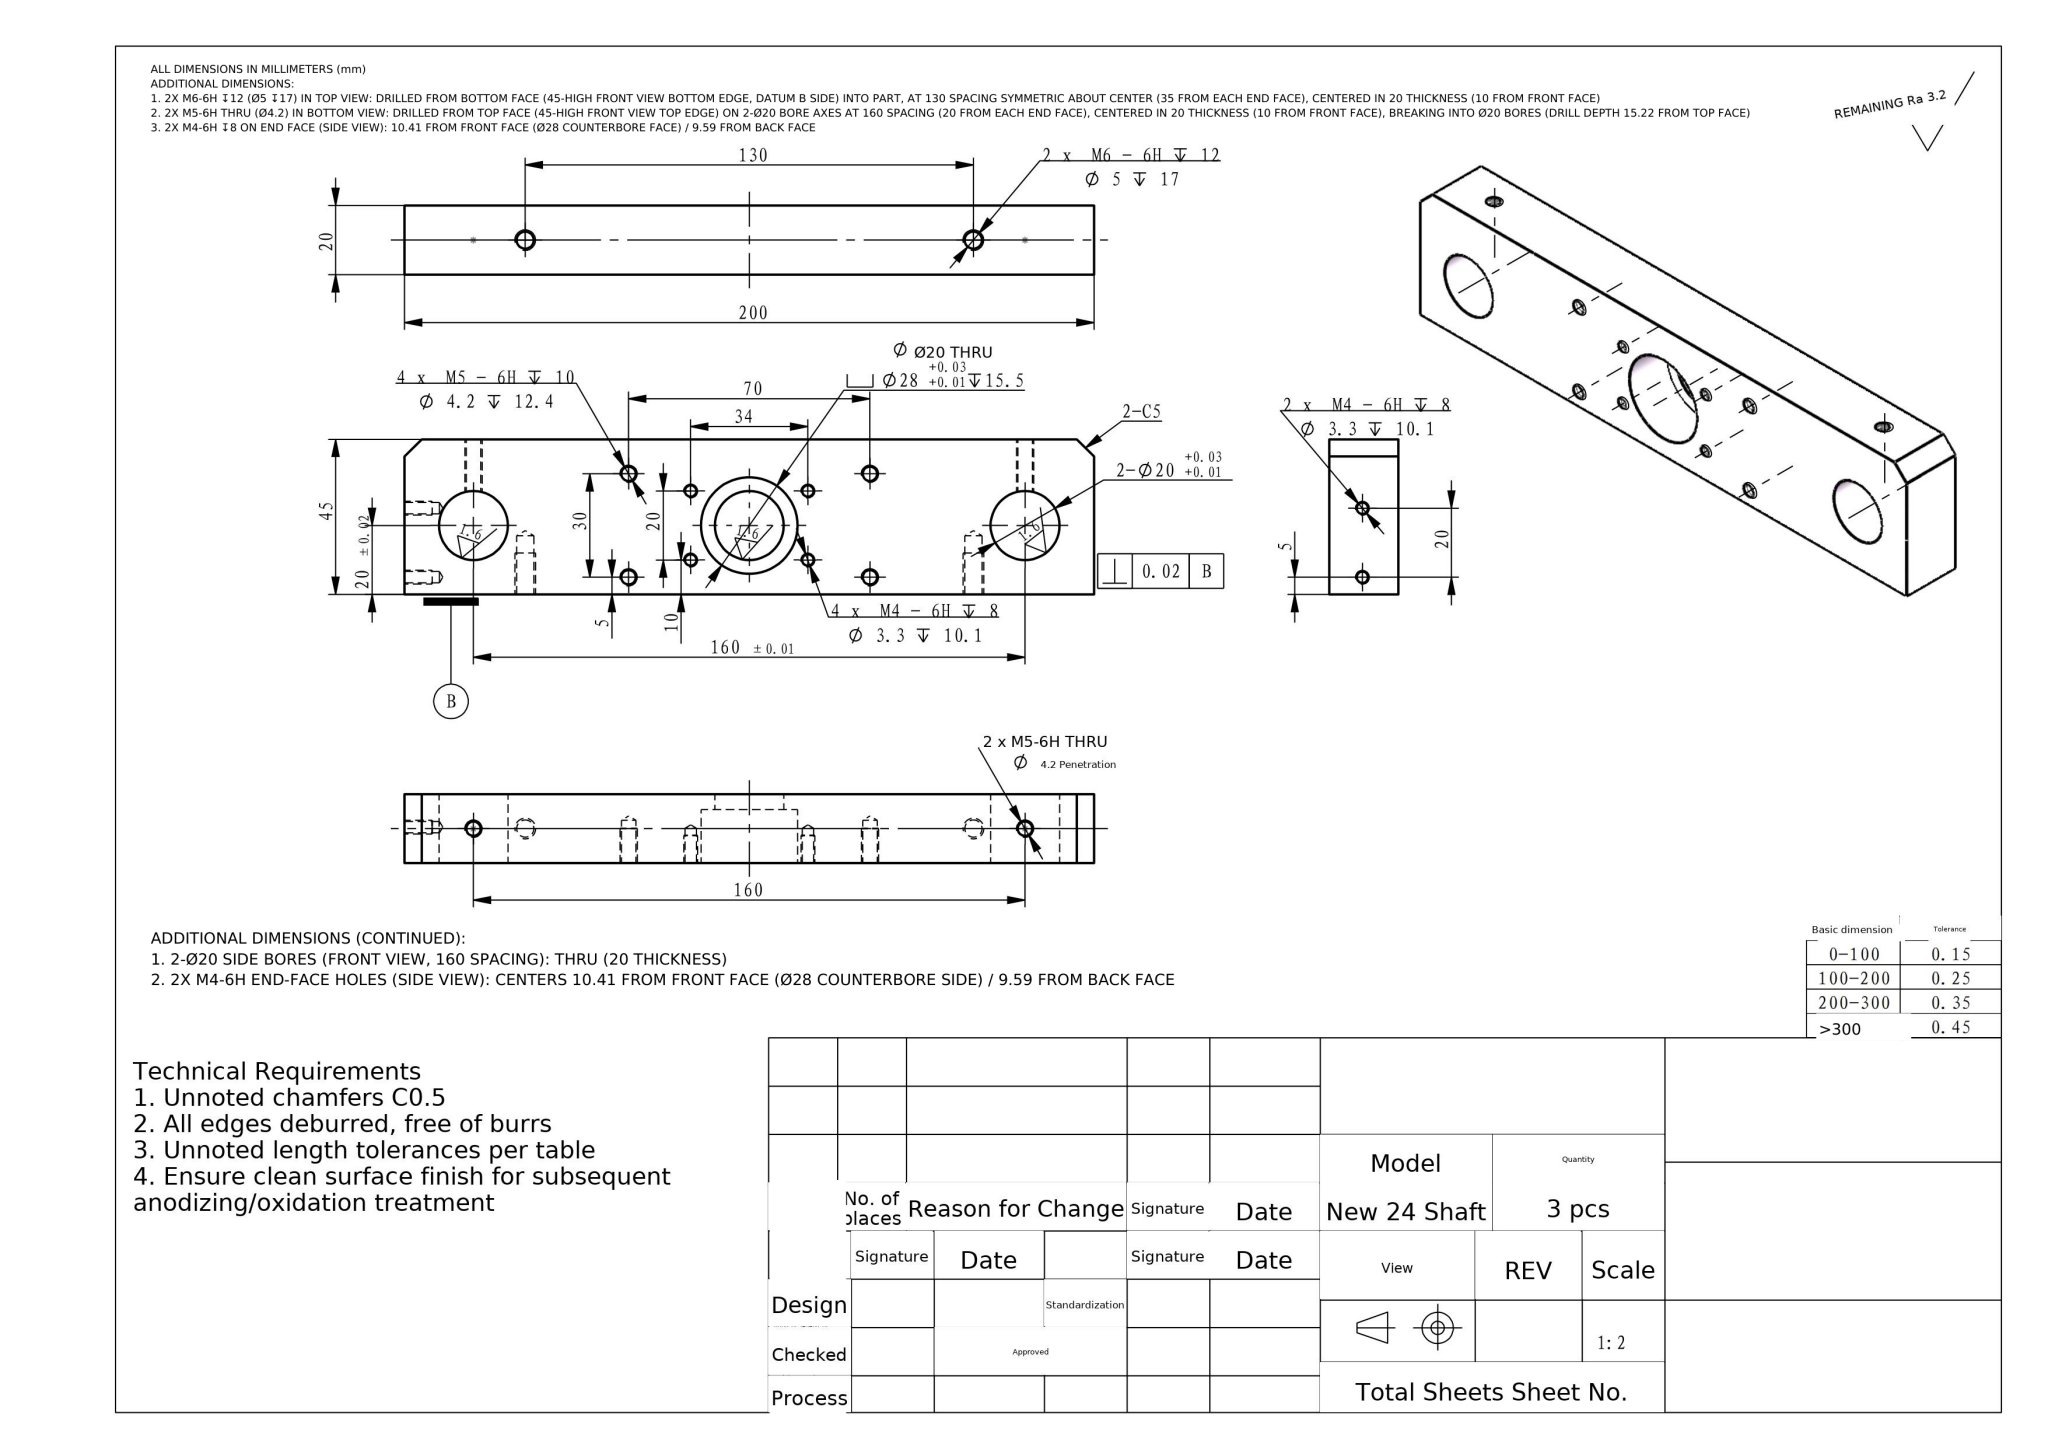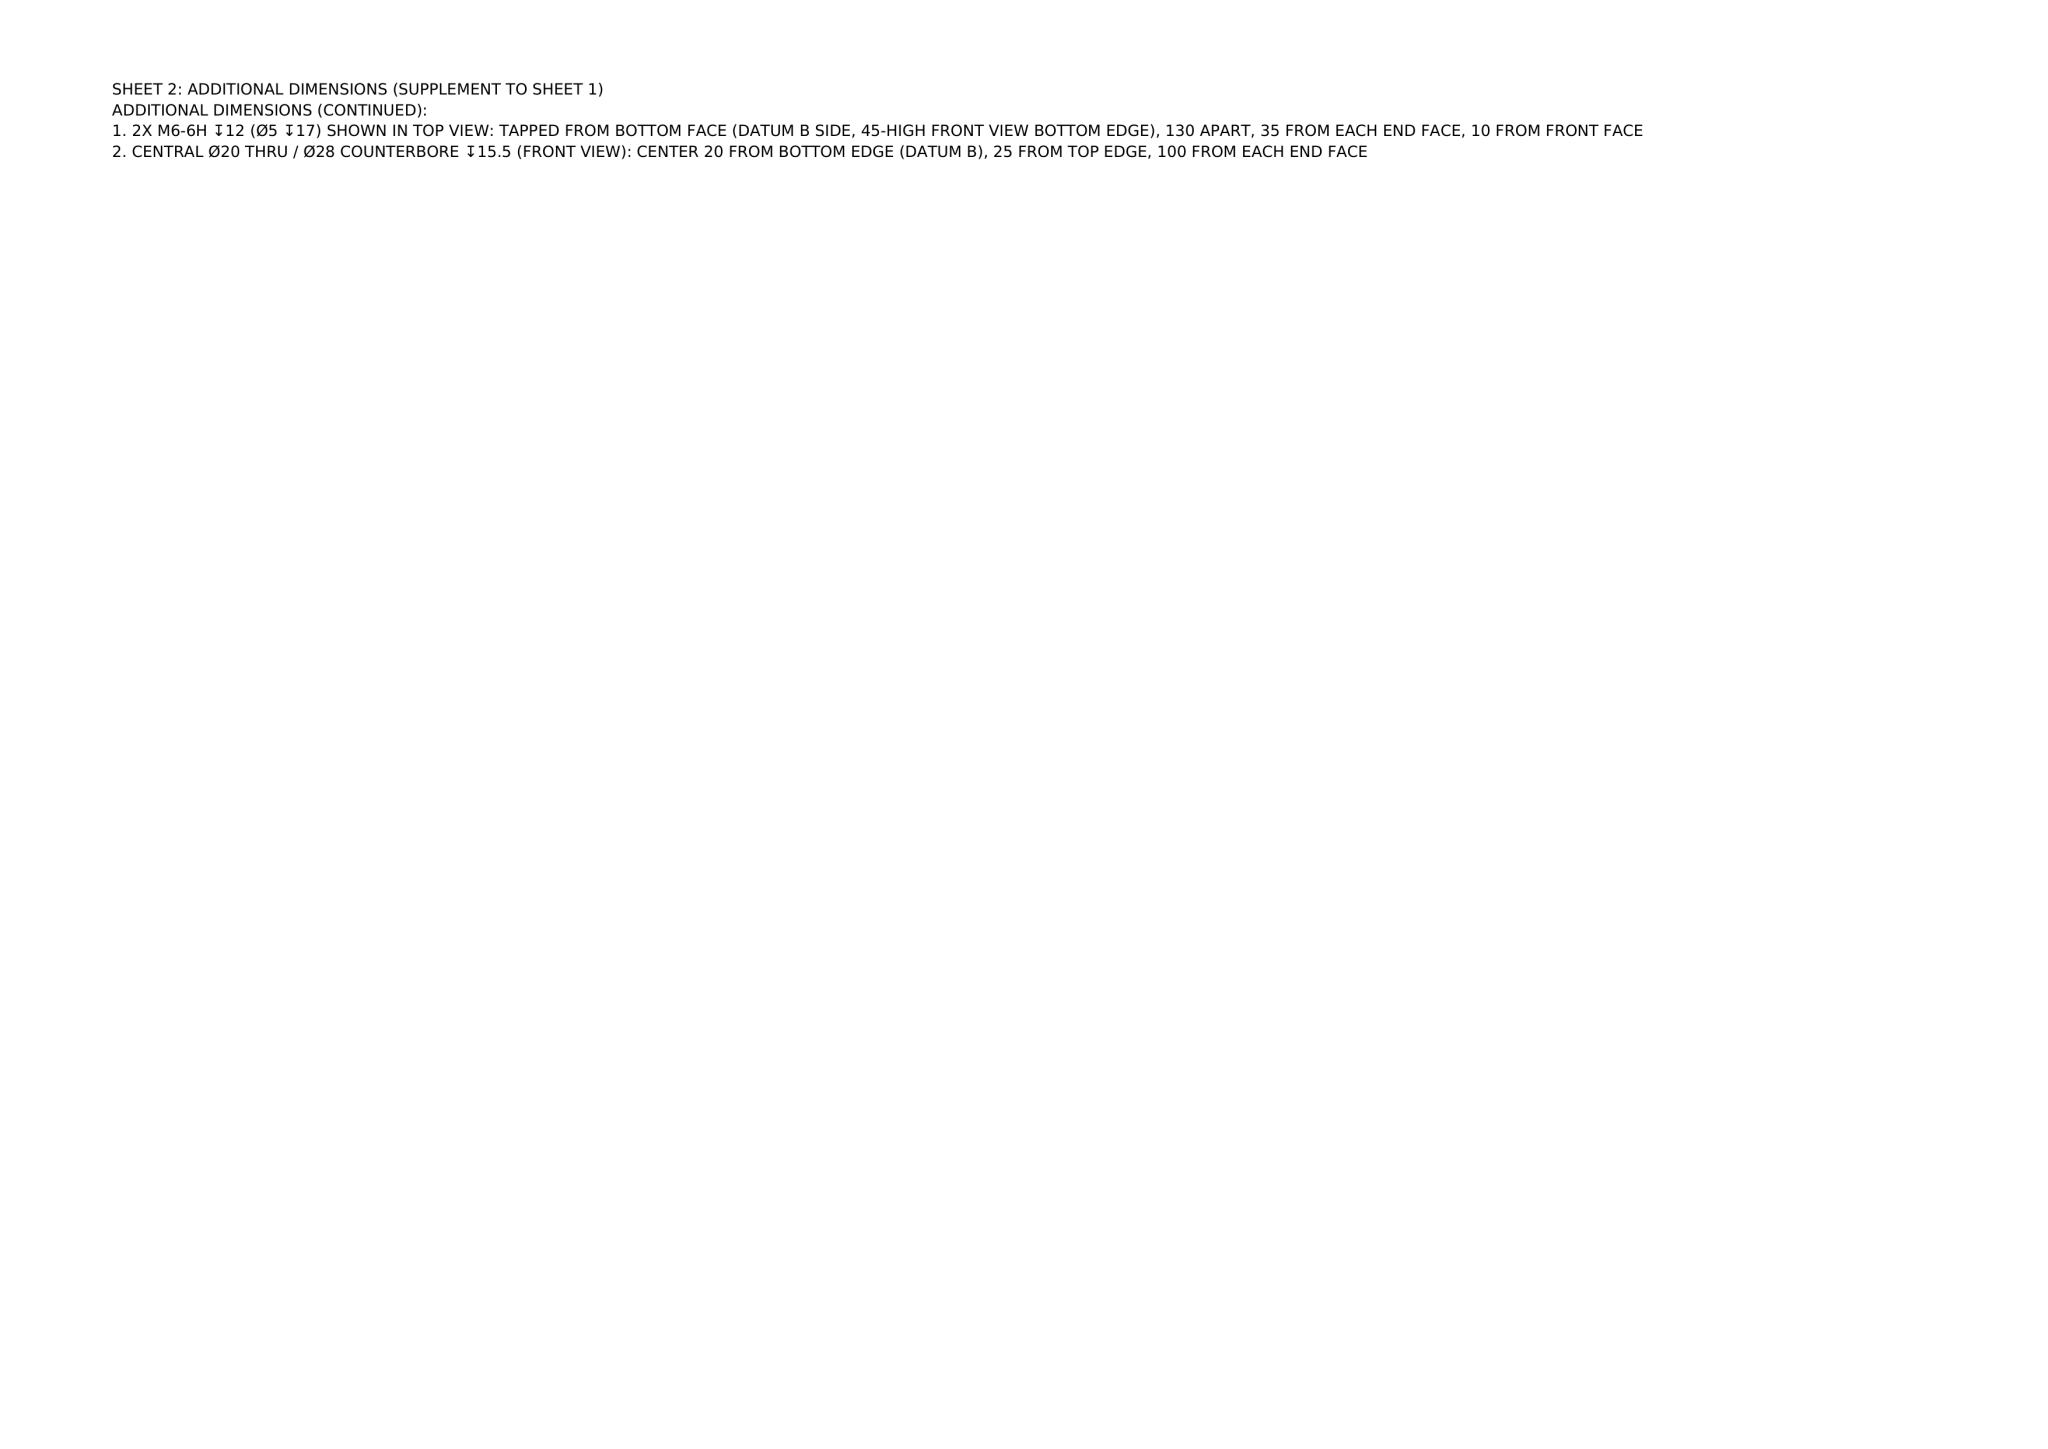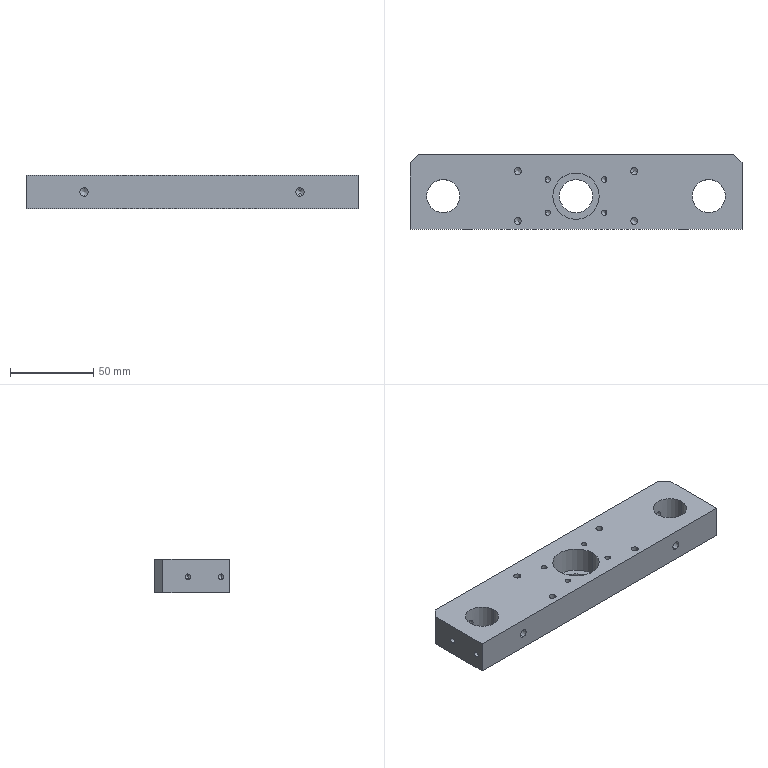Part | NX | mm | 1 solid | 69 faces | box 200 x 45 x 20 mm | volume 153626 mm3 | cylinder 36 | cone 24 | plane 9 | commonest cylinder face diameters 4.2 x12 3.3 x12 20 x6 5 x4 28 x2